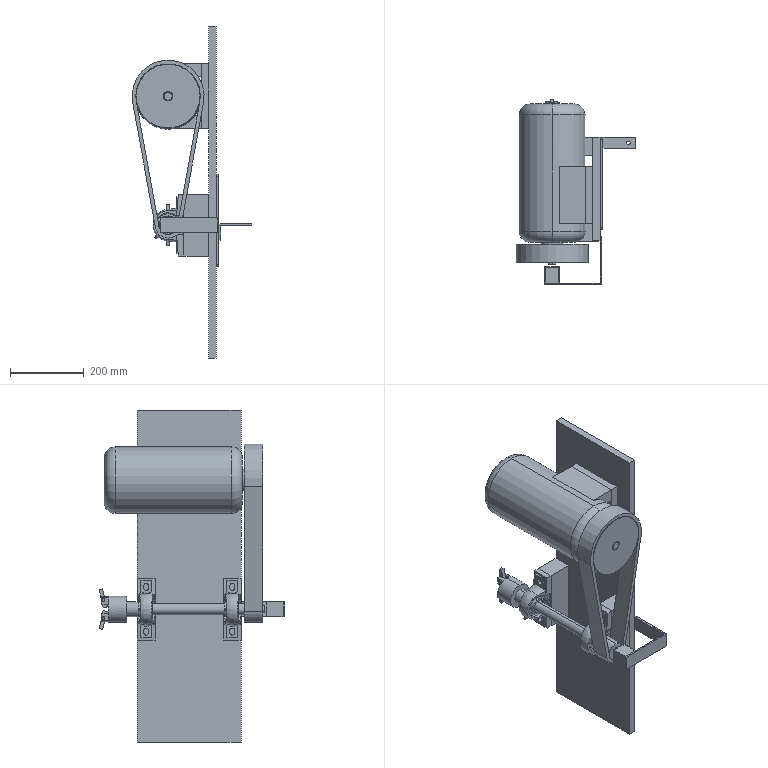Assembly | SolidWorks | mm | 19 component files | 20 solids | 579 faces | box 324.5 x 503.48 x 900 mm | volume 19296395 mm3 | plane 312 | cylinder 126 | cone 80 | torus 33 | sphere 16 | spline 12 | commonest cylinder face diameters 6 x16 10 x12 67.524 x12 39.28 x12 50.52 x12 13 x8 30 x6 8 x6
Bill of materials:
BasePlate | 1 | 45 | Thin flat rectangular plate, tall and narrow, with plain square edges.
BearingHousingBasePlate | 2 | 45 | Solid rectangular block (prism), taller than it is wide, with sharp edges.
Explosion-proofCasing | 1 | 45 | Short length of thin-walled square or near-square hollow tube, open at both ends.
FlipWindow | 1 | 45 | Thin flat plate, close to square, with small rounded corners and slightly softened edges.
GB_T7810-1995BearingUnitUCP206 | 2 |  | Housing with a rounded body and a central through bore holding a ring-shaped insert, attached to a rectangular base plate. The base plate has two slotted mounting holes, one in each end, set in recessed pads. Overall it looks like a pillow-block style bearing housing.
LargePulley | 1 | 45 | Solid round disc with a small concentric through hole, thick relative to the hole size, with small chamfered or rounded edges.
MotorBasePlate | 1 | 45 | Thick rectangular plate, close to square, with sharp edges and no visible features.
PressJaw | 2 | 45 | Rectangular bar set at an angle, with one round through hole, and an angled tapered tab sticking out sideways from one end to form a dog-leg or hook profile. Edges have small breaks.
PullPlate | 1 | 45 | L-shaped angle bracket with constant thickness: one short leg and one long leg. The long leg has a single round through hole near its rounded-corner free end.
RotatingShaft | 2 | 45 | Headed cylindrical pin: a long plain round shank with a short, larger-diameter head at one end and a flat or slightly chamfered tip at the other.
SensorHolder | 1 | 45 | L-shaped angle profile with thin, constant-thickness legs that look close to equal in length, extruded over a short length.
SmallPulley | 1 | 45 | Long slender rod-like body with stepped cylindrical sections. One end has a short larger cylinder with a small central boss. The other end has a stepped larger cylinder with two flat parallel tabs, each with a small hole. It looks like a multi-section turned shaft or rod assembly.
TimingBelt | 1 | Custom Plastic | Thin-walled closed band, teardrop-shaped in plan: a large rounded end tapering along straight sides to a small rounded end, extruded to a constant height with an open center.
Workpiece | 1 | 45 | Flanged cylindrical bushing-like solid: a short, larger-diameter disc flange joined coaxially to a longer, smaller-diameter cylindrical shank, with a small central round hole in the flange face.
YBBP-903-2-1.5Motor | 1 | 45 | Elongated cylindrical body with rounded/filleted ends. A small coaxial cylindrical shaft sticks out of one end, with a short collar/boss at its base. Two rectangular bar-like blocks run lengthwise along one side of the body, one above the other and parallel.
Mates:
1. coincident | YBBP-903-2-1.5Motor-1 face at (-383.359, -342.185, 1412) dir (0, -1, 0) | LargePulley-1 face at (-371.359, -342.185, 1412) dir (0, 1, 0)
2. concentric | YBBP-903-2-1.5Motor-1 face at (-371.359, -392.185, 1412) dir (0, -1, 0) r 12 | LargePulley-1 face at (-371.359, -392.185, 1412) dir (0, 1, 0) r 87.5
3. distance | SmallPulley-1 face at (-371.359, -342.185, 1062) dir (0, -1, 0) r 25 | LargePulley-1 face at (-371.359, -392.185, 1412) dir (0, 1, 0) r 87.5
4. concentric | LargePulley-1 face at (-371.359, -392.185, 1412) dir (0, 1, 0) r 87.5 | TimingBelt-1 face at (-371.359, -342.185, 1412) dir (0, -1, 0) r 87.5
5. coincident | LargePulley-1 face at (-371.359, -392.185, 1412) dir (0, -1, 0) | TimingBelt-1 face at (-371.359, -392.185, 1062) dir (0, -1, 0)
6. concentric | SmallPulley-1 face at (-371.359, -54.085, 1062) dir (0, -1, 0) r 15 | GB_T7810-1995BearingUnitUCP206-3 face at (-371.359, -76.285, 1062) dir (0, 1, 0) r 15
7. distance | SmallPulley-1 face at (-371.359, -342.185, 1062) dir (0, -1, 0) | GB_T7810-1995BearingUnitUCP206-3 face at (-390.999, -92.185, 1062) dir (0, -1, 0)
8. coincident | LargePulley-1 face at (-371.359, -392.185, 1412) dir (0, -1, 0) | SmallPulley-1 face at (-371.359, -392.185, 1062) dir (0, -1, 0)
9. coincident | GB_T7810-1995BearingUnitUCP206-3 face at (-328.459, -52.285, 1145.5) dir (0, 1, 0) | BasePlate-1 face at (-261.359, -52.285, 1602) dir (0, 1, 0)
10. coincident | BasePlate-1 face at (-261.359, -192.885, 1152) dir (-1, 0, 0) | MotorBasePlate-1 face at (-261.359, -208.685, 1412) dir (1, 0, 0)
11. coincident | YBBP-903-2-1.5Motor-1 face at (-500371.359, -131.185, 1324) dir (0, 0, -1) | MotorBasePlate-1 face at (-281.359, -286.185, 1324) dir (0, 0, -1)
12. coincident | YBBP-903-2-1.5Motor-1 face at (-500371.359, -131.185, 1324) dir (0, 1, 0) | MotorBasePlate-1 face at (-281.359, -131.185, 1500) dir (0, 1, 0)
13. coincident | BasePlate-1 face at (-261.359, -192.885, 1152) dir (-1, 0, 0) | BearingHousingBasePlate-1 face at (-261.359, -76.285, 1062) dir (1, 0, 0)
14. coincident | GB_T7810-1995BearingUnitUCP206-3 face at (-343.659, -52.285, 978.5) dir (0, 0, -1) | BearingHousingBasePlate-1 face at (-261.359, -100.285, 978.5) dir (0, 0, -1)
15. coincident | GB_T7810-1995BearingUnitUCP206-3 face at (-328.459, -52.285, 1035.846) dir (0, 1, 0) | BearingHousingBasePlate-1 face at (-261.359, -52.285, 978.5) dir (0, 1, 0)
16. coincident | BasePlate-1 face at (-261.359, -192.885, 1152) dir (-1, 0, 0) | BearingHousingBasePlate-2 face at (-261.359, -309.485, 1062) dir (1, 0, 0)
17. concentric | SmallPulley-1 face at (-371.359, 45.915, 1062) dir (0, -1, 0) r 35 | Workpiece-1 face at (-371.359, -10.905, 1062) dir (0, 1, 0) r 19.105
18. coincident | SmallPulley-1 face at (-371.359, -10.905, 1062) dir (0, 1, 0) | Workpiece-1 face at (-371.359, -10.905, 1062) dir (0, -1, 0)
19. parallel | GB_T7810-1995BearingUnitUCP206-3 face at (-343.659, -52.285, 1145.5) dir (0, 0, 1) | Workpiece-1 plane at (-371.359, -2.905, 1062) dir (0, 0, 1)
20. perpendicular | SmallPulley-1 face at (-386.359, 25.915, 1093.623) dir (-1, 0, 0) | BearingHousingBasePlate-1 face at (-261.359, -100.285, 1145.5) dir (0, 0, 1)
21. concentric | SmallPulley-1 face at (-406.359, 39.915, 1037.377) dir (1, 0, 0) r 3 | PressJaw-1 face at (-376.359, 39.915, 1037.377) dir (1, 0, 0) r 3
22. width | SmallPulley-1 face at (-364.359, -65.168, 1017) dir (-1, 0, 0) | SmallPulley-1 face at (-378.359, -65.168, 1017) dir (1, 0, 0) | PressJaw-1 face at (-366.359, 51.336, 1009.189) dir (1, 0, 0) | PressJaw-1 face at (-376.359, 51.336, 1009.189) dir (-1, 0, 0)
23. concentric | SmallPulley-1 face at (-406.359, 39.915, 1037.377) dir (1, 0, 0) r 3 | RotatingShaft-1 face at (-388.859, 39.915, 1037.377) dir (-1, 0, 0) r 3
24. coincident | SmallPulley-1 face at (-386.359, 25.915, 1093.623) dir (-1, 0, 0) | RotatingShaft-1 face at (-386.359, 43.915, 1037.377) dir (1, 0, 0)
25. coincident | FlipWindow-1 face at (-233.359, -177.285, 1075) dir (1, 0, 0) | PullPlate-1 face at (-233.359, -82.285, 1066) dir (-1, 0, 0)
26. coincident | BasePlate-1 face at (-241.359, -192.885, 1152) dir (1, 0, 0) | SensorHolder-1 face at (-241.359, -447.185, 1082) dir (-1, 0, 0)
27. distance | SensorHolder-1 face at (-391.359, -447.185, 1082) dir (0, 1, 0) | SmallPulley-1 face at (-371.359, -397.185, 1062) dir (0, -1, 0)
28. coincident | SensorHolder-1 face at (-391.359, -447.185, 1082) dir (0, 1, 0) | Explosion-proofCasing-1 face at (-371.359, -447.185, 1062) dir (0, -1, 0)
29. coincident | SensorHolder-1 face at (-391.359, -447.185, 1082) dir (0, 0, 1) | Explosion-proofCasing-1 edge at (-351.359, -447.185, 1082) dir (-1, 0, 0)
30. coincident | SensorHolder-1 face at (-391.359, -452.185, 1082) dir (-1, 0, 0) | Explosion-proofCasing-1 edge at (-391.359, -447.185, 1082) dir (0, 0, -1)
31. coincident | BasePlate-1 face at (-241.359, -192.885, 1152) dir (1, 0, 0) | FlipWindow-1 face at (-241.359, -177.285, 1075) dir (-1, 0, 0)
32. coincident | BasePlate-1 face at (-261.359, -52.285, 1602) dir (0, 1, 0) | FlipWindow-1 face at (-233.359, -52.285, 1200) dir (0, 1, 0)
33. coincident | FlipWindow-1 face at (-233.359, -52.285, 1200) dir (0, 1, 0) | PullPlate-1 face at (-228.359, -52.285, 1021) dir (0, 1, 0)